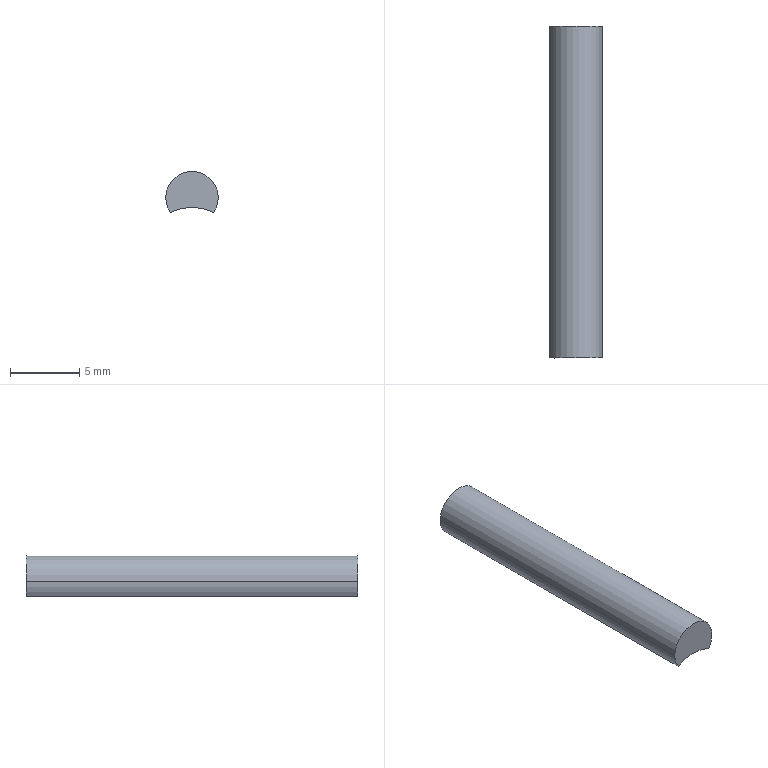Component | SolidWorks | SiliconeStrip3x24-1 | 1 solid | 6 faces | box 3.8 x 24 x 2.97 mm | volume 209 mm3 | cylinder 4 | plane 2 | commonest cylinder face diameters 3.8 x3 7 x1 | material Q235-A
build123d program:
from build123d import *

# Parameters (mm, degrees)
SKETCH1_2_R               = 1.9
BOSS_EXTRUDE1_DEPTH       = 12
SKETCH1_R                 = 3.5
ROLLERCONTACTRELIEF_DEPTH = 15


with BuildPart() as part:
    # Sketch1_2 → Boss-Extrude1 (new, symmetric)
    with BuildSketch(Plane.XY):
        Circle(SKETCH1_2_R)
    extrude(amount=BOSS_EXTRUDE1_DEPTH, both=True)

    # Sketch1 → RollerContactRelief (cut, symmetric)
    with BuildSketch(Plane.XY):
        with Locations((0, -4.2)):
            Circle(SKETCH1_R)
    extrude(amount=ROLLERCONTACTRELIEF_DEPTH, both=True, mode=Mode.SUBTRACT)


solid = part.part

# Placed as in the assembly
solid = solid.moved(Location((210.87, 43.668, 38.929), (90, 0, 0)))
STEP:
#1=CARTESIAN_POINT('',(8.377,1.247,1.533));
#2=VERTEX_POINT('',#1);
#3=CARTESIAN_POINT('',(8.227,1.247,1.533));
#4=VERTEX_POINT('',#3);
#5=CARTESIAN_POINT('',(8.302,1.247,1.533));
#6=DIRECTION('',(0.,-1.,0.));
#7=DIRECTION('',(1.,0.,0.));
#8=AXIS2_PLACEMENT_3D('',#5,#6,#7);
#9=CIRCLE('',#8,0.0748);
#10=EDGE_CURVE('',#2,#4,#9,.T.);
#11=ORIENTED_EDGE('',*,*,#10,.F.);
#12=CARTESIAN_POINT('',(8.377,2.192,1.533));
#13=VERTEX_POINT('',#12);
#14=CARTESIAN_POINT('',(8.377,1.247,1.533));
#15=DIRECTION('',(-0.,1.,-0.));
#16=VECTOR('',#15,39.37);
#17=LINE('',#14,#16);
#18=EDGE_CURVE('',#2,#13,#17,.T.);
#19=ORIENTED_EDGE('',*,*,#18,.T.);
#20=CARTESIAN_POINT('',(8.227,2.192,1.533));
#21=VERTEX_POINT('',#20);
#22=CARTESIAN_POINT('',(8.302,2.192,1.533));
#23=DIRECTION('',(0.,-1.,0.));
#24=DIRECTION('',(1.,0.,0.));
#25=AXIS2_PLACEMENT_3D('',#22,#23,#24);
#26=CIRCLE('',#25,0.0748);
#27=EDGE_CURVE('',#13,#21,#26,.T.);
#28=ORIENTED_EDGE('',*,*,#27,.T.);
#29=CARTESIAN_POINT('',(8.227,1.247,1.533));
#30=DIRECTION('',(-0.,1.,-0.));
#31=VECTOR('',#30,39.37);
#32=LINE('',#29,#31);
#33=EDGE_CURVE('',#4,#21,#32,.T.);
#34=ORIENTED_EDGE('',*,*,#33,.F.);
#35=EDGE_LOOP('',(#11,#19,#28,#34));
#36=FACE_OUTER_BOUND('',#35,.T.);
#37=CARTESIAN_POINT('',(8.302,1.247,1.533));
#38=DIRECTION('',(-0.,1.,-0.));
#39=DIRECTION('',(-1.,0.,0.));
#40=AXIS2_PLACEMENT_3D('',#37,#38,#39);
#41=CYLINDRICAL_SURFACE('',#40,0.0748);
#42=ADVANCED_FACE('',(#36),#41,.T.);
#43=CARTESIAN_POINT('',(8.24,1.247,1.49));
#44=VERTEX_POINT('',#43);
#45=CARTESIAN_POINT('',(8.302,1.247,1.533));
#46=DIRECTION('',(0.,-1.,0.));
#47=DIRECTION('',(1.,0.,0.));
#48=AXIS2_PLACEMENT_3D('',#45,#46,#47);
#49=CIRCLE('',#48,0.0748);
#50=EDGE_CURVE('',#4,#44,#49,.T.);
#51=ORIENTED_EDGE('',*,*,#50,.F.);
#52=ORIENTED_EDGE('',*,*,#33,.T.);
#53=CARTESIAN_POINT('',(8.24,2.192,1.49));
#54=VERTEX_POINT('',#53);
#55=CARTESIAN_POINT('',(8.302,2.192,1.533));
#56=DIRECTION('',(0.,-1.,0.));
#57=DIRECTION('',(1.,0.,0.));
#58=AXIS2_PLACEMENT_3D('',#55,#56,#57);
#59=CIRCLE('',#58,0.0748);
#60=EDGE_CURVE('',#21,#54,#59,.T.);
#61=ORIENTED_EDGE('',*,*,#60,.T.);
#62=CARTESIAN_POINT('',(8.24,1.719,1.49));
#63=DIRECTION('',(0.,-1.,0.));
#64=VECTOR('',#63,39.37);
#65=LINE('',#62,#64);
#66=EDGE_CURVE('',#54,#44,#65,.T.);
#67=ORIENTED_EDGE('',*,*,#66,.T.);
#68=EDGE_LOOP('',(#51,#52,#61,#67));
#69=FACE_OUTER_BOUND('',#68,.T.);
#70=CARTESIAN_POINT('',(8.302,1.247,1.533));
#71=DIRECTION('',(-0.,1.,-0.));
#72=DIRECTION('',(-1.,0.,0.));
#73=AXIS2_PLACEMENT_3D('',#70,#71,#72);
#74=CYLINDRICAL_SURFACE('',#73,0.0748);
#75=ADVANCED_FACE('',(#69),#74,.T.);
#76=ORIENTED_EDGE('',*,*,#18,.F.);
#77=CARTESIAN_POINT('',(8.364,1.247,1.49));
#78=VERTEX_POINT('',#77);
#79=CARTESIAN_POINT('',(8.302,1.247,1.533));
#80=DIRECTION('',(0.,-1.,0.));
#81=DIRECTION('',(1.,0.,0.));
#82=AXIS2_PLACEMENT_3D('',#79,#80,#81);
#83=CIRCLE('',#82,0.0748);
#84=EDGE_CURVE('',#78,#2,#83,.T.);
#85=ORIENTED_EDGE('',*,*,#84,.F.);
#86=CARTESIAN_POINT('',(8.364,2.192,1.49));
#87=VERTEX_POINT('',#86);
#88=CARTESIAN_POINT('',(8.364,1.719,1.49));
#89=DIRECTION('',(-0.,1.,-0.));
#90=VECTOR('',#89,39.37);
#91=LINE('',#88,#90);
#92=EDGE_CURVE('',#78,#87,#91,.T.);
#93=ORIENTED_EDGE('',*,*,#92,.T.);
#94=CARTESIAN_POINT('',(8.302,2.192,1.533));
#95=DIRECTION('',(0.,-1.,0.));
#96=DIRECTION('',(1.,0.,0.));
#97=AXIS2_PLACEMENT_3D('',#94,#95,#96);
#98=CIRCLE('',#97,0.0748);
#99=EDGE_CURVE('',#87,#13,#98,.T.);
#100=ORIENTED_EDGE('',*,*,#99,.T.);
#101=EDGE_LOOP('',(#76,#85,#93,#100));
#102=FACE_OUTER_BOUND('',#101,.T.);
#103=CARTESIAN_POINT('',(8.302,1.247,1.533));
#104=DIRECTION('',(-0.,1.,-0.));
#105=DIRECTION('',(-1.,0.,0.));
#106=AXIS2_PLACEMENT_3D('',#103,#104,#105);
#107=CYLINDRICAL_SURFACE('',#106,0.0748);
#108=ADVANCED_FACE('',(#102),#107,.T.);
#109=CARTESIAN_POINT('',(8.302,1.247,1.367));
#110=DIRECTION('',(0.,-1.,0.));
#111=DIRECTION('',(1.,0.,-0.));
#112=AXIS2_PLACEMENT_3D('',#109,#110,#111);
#113=CIRCLE('',#112,0.1378);
#114=EDGE_CURVE('',#78,#44,#113,.T.);
#115=ORIENTED_EDGE('',*,*,#114,.F.);
#116=ORIENTED_EDGE('',*,*,#84,.T.);
#117=ORIENTED_EDGE('',*,*,#10,.T.);
#118=ORIENTED_EDGE('',*,*,#50,.T.);
#119=EDGE_LOOP('',(#115,#116,#117,#118));
#120=FACE_OUTER_BOUND('',#119,.T.);
#121=CARTESIAN_POINT('',(8.302,1.247,1.533));
#122=DIRECTION('',(0.,-1.,0.));
#123=DIRECTION('',(1.,0.,-0.));
#124=AXIS2_PLACEMENT_3D('',#121,#122,#123);
#125=PLANE('',#124);
#126=ADVANCED_FACE('',(#120),#125,.T.);
#127=ORIENTED_EDGE('',*,*,#99,.F.);
#128=CARTESIAN_POINT('',(8.302,2.192,1.367));
#129=DIRECTION('',(0.,-1.,0.));
#130=DIRECTION('',(1.,0.,-0.));
#131=AXIS2_PLACEMENT_3D('',#128,#129,#130);
#132=CIRCLE('',#131,0.1378);
#133=EDGE_CURVE('',#87,#54,#132,.T.);
#134=ORIENTED_EDGE('',*,*,#133,.T.);
#135=ORIENTED_EDGE('',*,*,#60,.F.);
#136=ORIENTED_EDGE('',*,*,#27,.F.);
#137=EDGE_LOOP('',(#127,#134,#135,#136));
#138=FACE_OUTER_BOUND('',#137,.T.);
#139=CARTESIAN_POINT('',(8.302,2.192,1.533));
#140=DIRECTION('',(0.,-1.,0.));
#141=DIRECTION('',(1.,0.,-0.));
#142=AXIS2_PLACEMENT_3D('',#139,#140,#141);
#143=PLANE('',#142);
#144=ADVANCED_FACE('',(#138),#143,.F.);
#145=ORIENTED_EDGE('',*,*,#114,.T.);
#146=ORIENTED_EDGE('',*,*,#66,.F.);
#147=ORIENTED_EDGE('',*,*,#133,.F.);
#148=ORIENTED_EDGE('',*,*,#92,.F.);
#149=EDGE_LOOP('',(#145,#146,#147,#148));
#150=FACE_OUTER_BOUND('',#149,.T.);
#151=CARTESIAN_POINT('',(8.302,2.31,1.367));
#152=DIRECTION('',(0.,-1.,0.));
#153=DIRECTION('',(1.,0.,-0.));
#154=AXIS2_PLACEMENT_3D('',#151,#152,#153);
#155=CYLINDRICAL_SURFACE('',#154,0.1378);
#156=ADVANCED_FACE('',(#150),#155,.F.);
#157=CLOSED_SHELL('',(#42,#75,#108,#126,#144,#156));
#158=MANIFOLD_SOLID_BREP('',#157);
#159=CARTESIAN_POINT('',(0.,0.,0.));
#160=DIRECTION('',(0.,0.,1.));
#161=DIRECTION('',(1.,0.,0.));
#162=AXIS2_PLACEMENT_3D('',#159,#160,#161);
#163=(LENGTH_UNIT()NAMED_UNIT(*)SI_UNIT($,.METRE.));
#164=LENGTH_MEASURE_WITH_UNIT(LENGTH_MEASURE(0.0254),#163);
#165=DIMENSIONAL_EXPONENTS(1.,0.,0.,0.,0.,0.,0.);
#166=(CONVERSION_BASED_UNIT('',#164)LENGTH_UNIT()NAMED_UNIT(#165));
#167=UNCERTAINTY_MEASURE_WITH_UNIT(LENGTH_MEASURE(0.00001),#166,'','');
#168=(NAMED_UNIT(*)PLANE_ANGLE_UNIT()SI_UNIT($,.RADIAN.));
#169=(NAMED_UNIT(*)SI_UNIT($,.STERADIAN.)SOLID_ANGLE_UNIT());
#170=(GEOMETRIC_REPRESENTATION_CONTEXT(3)GLOBAL_UNCERTAINTY_ASSIGNED_CONTEXT((#167))GLOBAL_UNIT_ASSIGNED_CONTEXT((#166,#168,#169))REPRESENTATION_CONTEXT('',''));
#171=ADVANCED_BREP_SHAPE_REPRESENTATION('',(#158,#162),#170);
#172=COLOUR_RGB('',0.7922,0.8196,0.9333);
#173=FILL_AREA_STYLE_COLOUR('',#172);
#174=FILL_AREA_STYLE('',(#173));
#175=SURFACE_STYLE_FILL_AREA(#174);
#176=SURFACE_SIDE_STYLE('',(#175));
#177=SURFACE_STYLE_USAGE(.BOTH.,#176);
#178=PRESENTATION_STYLE_ASSIGNMENT((#177));
#179=STYLED_ITEM('',(#178),#158);
#180=(LENGTH_UNIT()NAMED_UNIT(*)SI_UNIT($,.METRE.));
#181=LENGTH_MEASURE_WITH_UNIT(LENGTH_MEASURE(0.0254),#180);
#182=DIMENSIONAL_EXPONENTS(1.,0.,0.,0.,0.,0.,0.);
#183=(CONVERSION_BASED_UNIT('',#181)LENGTH_UNIT()NAMED_UNIT(#182));
#184=UNCERTAINTY_MEASURE_WITH_UNIT(LENGTH_MEASURE(0.00001),#183,'','');
#185=(NAMED_UNIT(*)PLANE_ANGLE_UNIT()SI_UNIT($,.RADIAN.));
#186=(NAMED_UNIT(*)SI_UNIT($,.STERADIAN.)SOLID_ANGLE_UNIT());
#187=(GEOMETRIC_REPRESENTATION_CONTEXT(3)GLOBAL_UNCERTAINTY_ASSIGNED_CONTEXT((#184))GLOBAL_UNIT_ASSIGNED_CONTEXT((#183,#185,#186))REPRESENTATION_CONTEXT('',''));
#188=MECHANICAL_DESIGN_GEOMETRIC_PRESENTATION_REPRESENTATION('',(#179),#187);
#189=PRESENTATION_LAYER_ASSIGNMENT('','',(#179));